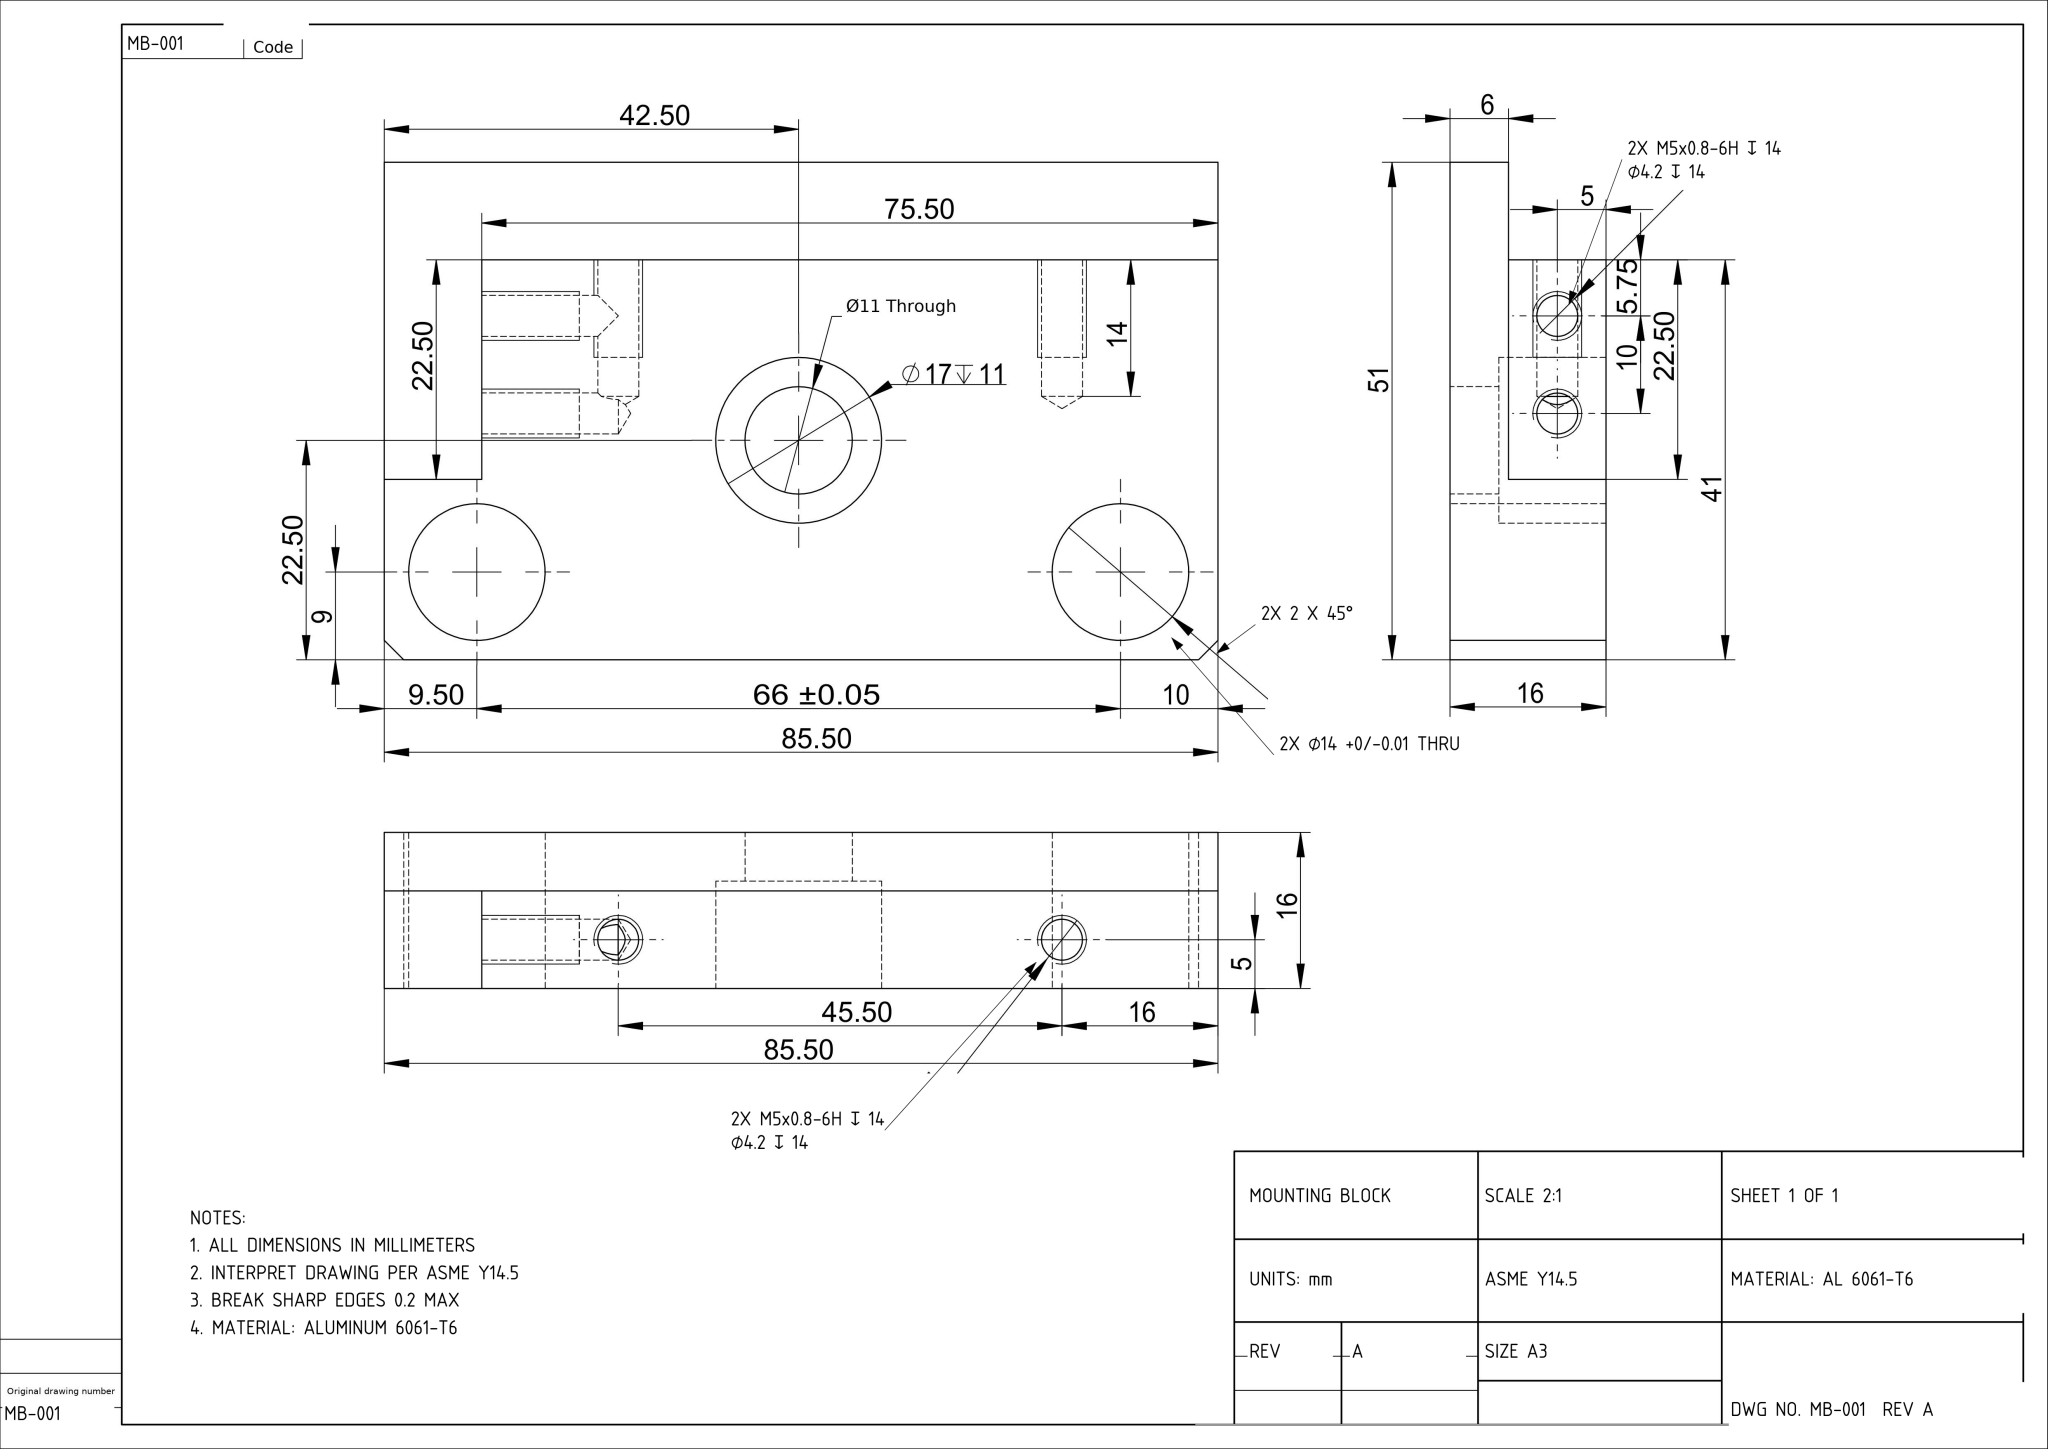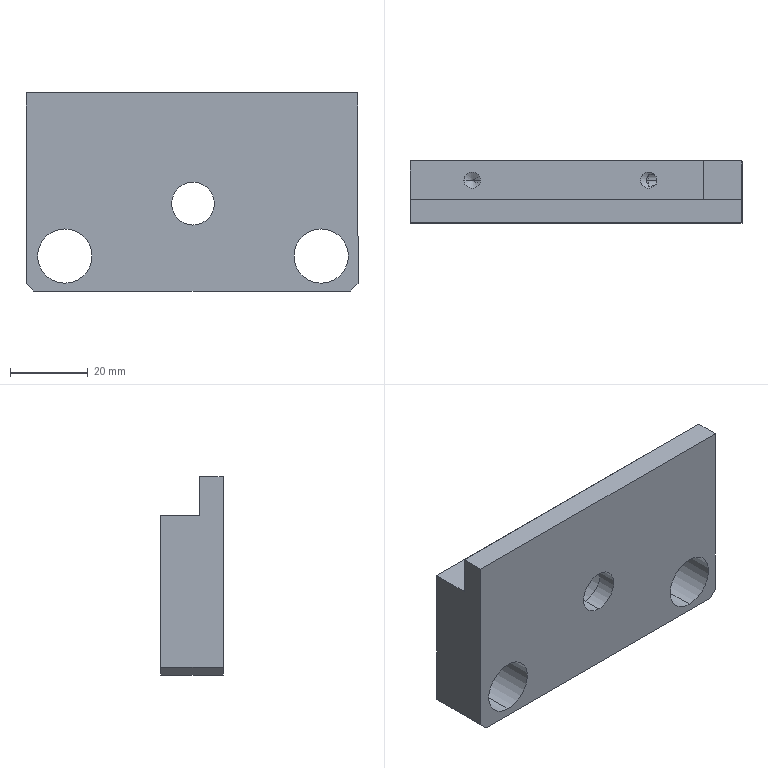Part | NX | mm | 1 solid | 34 faces | box 85.5 x 16 x 51 mm | volume 50242 mm3 | cylinder 16 | plane 13 | cone 5 | commonest cylinder face diameters 4.2 x8 14 x4 17 x2 11 x2